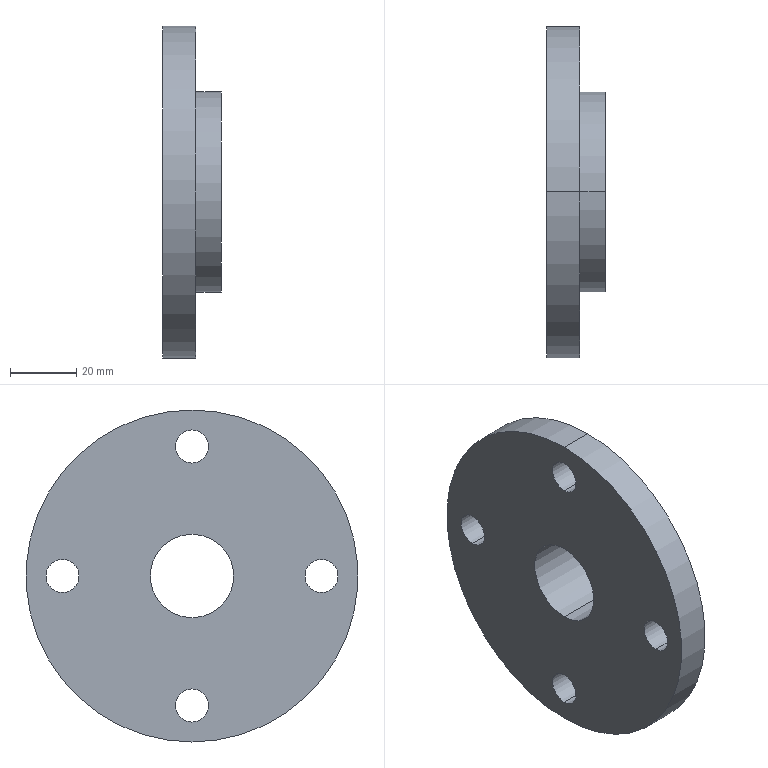Component | SolidWorks | FrontEndCap-1 | 1 solid | 17 faces | box 17.71 x 100 x 100 mm | volume 88740 mm3 | cylinder 14 | plane 3 | commonest cylinder face diameters 10 x8 25.135 x2 60.457 x2 100 x2
build123d program:
from build123d import *

# Parameters (mm, degrees)
SKETCH3_R          = 5
CUT_EXTRUDE1_DEPTH = 10


with BuildPart() as part:
    # Sketch2 → Revolve1 (revolve)
    with BuildSketch(Plane.ZY.offset(15), mode=Mode.PRIVATE) as revolve1_sk:
        Polygon((12.303, 200), (2.303, 200), (2.303, 180.229), (-5.405, 180.229), (-5.405, 162.567), (12.303, 162.567), align=None)
    revolve(revolve1_sk.sketch.rotate(Axis((-15, 150, 63.319), (0, 0, -1)), 90), axis=Axis((-15, 150, 63.319), (0, 0, -1)))

    # Sketch3 → Cut-Extrude1 (cut)
    with BuildSketch(Plane.XY.offset(12.303)):
        with Locations((24, 150)):
            Circle(SKETCH3_R)
        with Locations((-15, 111)):
            Circle(SKETCH3_R)
        with Locations((-54, 150)):
            Circle(SKETCH3_R)
        with Locations((-15, 189)):
            Circle(SKETCH3_R)
    extrude(amount=-CUT_EXTRUDE1_DEPTH, mode=Mode.SUBTRACT)


solid = part.part

# Placed as in the assembly
solid = solid.moved(Location((-122.697, 0, 0), (0, -90, 0)))
STEP:
#1=COLOUR_RGB('',0.7922,0.8196,0.9333);
#2=FILL_AREA_STYLE_COLOUR('',#1);
#3=FILL_AREA_STYLE('',(#2));
#4=SURFACE_STYLE_FILL_AREA(#3);
#5=SURFACE_SIDE_STYLE('',(#4));
#6=SURFACE_STYLE_USAGE(.BOTH.,#5);
#7=PRESENTATION_STYLE_ASSIGNMENT((#6));
#8=CARTESIAN_POINT('',(-4.921,5.906,0.748));
#9=VERTEX_POINT('',#8);
#10=CARTESIAN_POINT('',(-4.921,5.906,1.142));
#11=VERTEX_POINT('',#10);
#12=CARTESIAN_POINT('',(-4.921,5.906,0.9449));
#13=DIRECTION('',(-1.,0.,0.));
#14=DIRECTION('',(0.,0.,1.));
#15=AXIS2_PLACEMENT_3D('',#12,#13,#14);
#16=CIRCLE('',#15,0.1969);
#17=EDGE_CURVE('',#9,#11,#16,.T.);
#18=ORIENTED_EDGE('',*,*,#17,.F.);
#19=CARTESIAN_POINT('',(-5.315,5.906,0.748));
#20=VERTEX_POINT('',#19);
#21=CARTESIAN_POINT('',(-4.921,5.906,0.748));
#22=DIRECTION('',(-1.,0.,0.));
#23=VECTOR('',#22,39.37);
#24=LINE('',#21,#23);
#25=EDGE_CURVE('',#9,#20,#24,.T.);
#26=ORIENTED_EDGE('',*,*,#25,.T.);
#27=CARTESIAN_POINT('',(-5.315,5.906,1.142));
#28=VERTEX_POINT('',#27);
#29=CARTESIAN_POINT('',(-5.315,5.906,0.9449));
#30=DIRECTION('',(-1.,0.,0.));
#31=DIRECTION('',(0.,0.,1.));
#32=AXIS2_PLACEMENT_3D('',#29,#30,#31);
#33=CIRCLE('',#32,0.1969);
#34=EDGE_CURVE('',#20,#28,#33,.T.);
#35=ORIENTED_EDGE('',*,*,#34,.T.);
#36=CARTESIAN_POINT('',(-4.921,5.906,1.142));
#37=DIRECTION('',(-1.,0.,0.));
#38=VECTOR('',#37,39.37);
#39=LINE('',#36,#38);
#40=EDGE_CURVE('',#11,#28,#39,.T.);
#41=ORIENTED_EDGE('',*,*,#40,.F.);
#42=EDGE_LOOP('',(#18,#26,#35,#41));
#43=FACE_OUTER_BOUND('',#42,.T.);
#44=CARTESIAN_POINT('',(-4.921,5.906,0.9449));
#45=DIRECTION('',(-1.,0.,0.));
#46=DIRECTION('',(0.,0.,1.));
#47=AXIS2_PLACEMENT_3D('',#44,#45,#46);
#48=CYLINDRICAL_SURFACE('',#47,0.1969);
#49=ADVANCED_FACE('',(#43),#48,.F.);
#50=CARTESIAN_POINT('',(-4.921,4.37,-0.7874));
#51=VERTEX_POINT('',#50);
#52=CARTESIAN_POINT('',(-4.921,4.37,-0.3937));
#53=VERTEX_POINT('',#52);
#54=CARTESIAN_POINT('',(-4.921,4.37,-0.5906));
#55=DIRECTION('',(-1.,0.,0.));
#56=DIRECTION('',(0.,0.,1.));
#57=AXIS2_PLACEMENT_3D('',#54,#55,#56);
#58=CIRCLE('',#57,0.1969);
#59=EDGE_CURVE('',#51,#53,#58,.T.);
#60=ORIENTED_EDGE('',*,*,#59,.F.);
#61=CARTESIAN_POINT('',(-5.315,4.37,-0.7874));
#62=VERTEX_POINT('',#61);
#63=CARTESIAN_POINT('',(-4.921,4.37,-0.7874));
#64=DIRECTION('',(-1.,0.,0.));
#65=VECTOR('',#64,39.37);
#66=LINE('',#63,#65);
#67=EDGE_CURVE('',#51,#62,#66,.T.);
#68=ORIENTED_EDGE('',*,*,#67,.T.);
#69=CARTESIAN_POINT('',(-5.315,4.37,-0.3937));
#70=VERTEX_POINT('',#69);
#71=CARTESIAN_POINT('',(-5.315,4.37,-0.5906));
#72=DIRECTION('',(-1.,0.,0.));
#73=DIRECTION('',(0.,0.,1.));
#74=AXIS2_PLACEMENT_3D('',#71,#72,#73);
#75=CIRCLE('',#74,0.1969);
#76=EDGE_CURVE('',#62,#70,#75,.T.);
#77=ORIENTED_EDGE('',*,*,#76,.T.);
#78=CARTESIAN_POINT('',(-4.921,4.37,-0.3937));
#79=DIRECTION('',(-1.,0.,0.));
#80=VECTOR('',#79,39.37);
#81=LINE('',#78,#80);
#82=EDGE_CURVE('',#53,#70,#81,.T.);
#83=ORIENTED_EDGE('',*,*,#82,.F.);
#84=EDGE_LOOP('',(#60,#68,#77,#83));
#85=FACE_OUTER_BOUND('',#84,.T.);
#86=CARTESIAN_POINT('',(-4.921,4.37,-0.5906));
#87=DIRECTION('',(-1.,0.,0.));
#88=DIRECTION('',(0.,0.,1.));
#89=AXIS2_PLACEMENT_3D('',#86,#87,#88);
#90=CYLINDRICAL_SURFACE('',#89,0.1969);
#91=ADVANCED_FACE('',(#85),#90,.F.);
#92=CARTESIAN_POINT('',(-4.921,5.906,-2.323));
#93=VERTEX_POINT('',#92);
#94=CARTESIAN_POINT('',(-4.921,5.906,-1.929));
#95=VERTEX_POINT('',#94);
#96=CARTESIAN_POINT('',(-4.921,5.906,-2.126));
#97=DIRECTION('',(-1.,0.,0.));
#98=DIRECTION('',(0.,0.,1.));
#99=AXIS2_PLACEMENT_3D('',#96,#97,#98);
#100=CIRCLE('',#99,0.1969);
#101=EDGE_CURVE('',#93,#95,#100,.T.);
#102=ORIENTED_EDGE('',*,*,#101,.F.);
#103=CARTESIAN_POINT('',(-5.315,5.906,-2.323));
#104=VERTEX_POINT('',#103);
#105=CARTESIAN_POINT('',(-4.921,5.906,-2.323));
#106=DIRECTION('',(-1.,0.,0.));
#107=VECTOR('',#106,39.37);
#108=LINE('',#105,#107);
#109=EDGE_CURVE('',#93,#104,#108,.T.);
#110=ORIENTED_EDGE('',*,*,#109,.T.);
#111=CARTESIAN_POINT('',(-5.315,5.906,-1.929));
#112=VERTEX_POINT('',#111);
#113=CARTESIAN_POINT('',(-5.315,5.906,-2.126));
#114=DIRECTION('',(-1.,0.,0.));
#115=DIRECTION('',(0.,0.,1.));
#116=AXIS2_PLACEMENT_3D('',#113,#114,#115);
#117=CIRCLE('',#116,0.1969);
#118=EDGE_CURVE('',#104,#112,#117,.T.);
#119=ORIENTED_EDGE('',*,*,#118,.T.);
#120=CARTESIAN_POINT('',(-4.921,5.906,-1.929));
#121=DIRECTION('',(-1.,0.,0.));
#122=VECTOR('',#121,39.37);
#123=LINE('',#120,#122);
#124=EDGE_CURVE('',#95,#112,#123,.T.);
#125=ORIENTED_EDGE('',*,*,#124,.F.);
#126=EDGE_LOOP('',(#102,#110,#119,#125));
#127=FACE_OUTER_BOUND('',#126,.T.);
#128=CARTESIAN_POINT('',(-4.921,5.906,-2.126));
#129=DIRECTION('',(-1.,0.,0.));
#130=DIRECTION('',(0.,0.,1.));
#131=AXIS2_PLACEMENT_3D('',#128,#129,#130);
#132=CYLINDRICAL_SURFACE('',#131,0.1969);
#133=ADVANCED_FACE('',(#127),#132,.F.);
#134=CARTESIAN_POINT('',(-4.921,7.441,-0.7874));
#135=VERTEX_POINT('',#134);
#136=CARTESIAN_POINT('',(-4.921,7.441,-0.3937));
#137=VERTEX_POINT('',#136);
#138=CARTESIAN_POINT('',(-4.921,7.441,-0.5906));
#139=DIRECTION('',(-1.,0.,0.));
#140=DIRECTION('',(0.,0.,1.));
#141=AXIS2_PLACEMENT_3D('',#138,#139,#140);
#142=CIRCLE('',#141,0.1969);
#143=EDGE_CURVE('',#135,#137,#142,.T.);
#144=ORIENTED_EDGE('',*,*,#143,.F.);
#145=CARTESIAN_POINT('',(-5.315,7.441,-0.7874));
#146=VERTEX_POINT('',#145);
#147=CARTESIAN_POINT('',(-4.921,7.441,-0.7874));
#148=DIRECTION('',(-1.,0.,0.));
#149=VECTOR('',#148,39.37);
#150=LINE('',#147,#149);
#151=EDGE_CURVE('',#135,#146,#150,.T.);
#152=ORIENTED_EDGE('',*,*,#151,.T.);
#153=CARTESIAN_POINT('',(-5.315,7.441,-0.3937));
#154=VERTEX_POINT('',#153);
#155=CARTESIAN_POINT('',(-5.315,7.441,-0.5906));
#156=DIRECTION('',(-1.,0.,0.));
#157=DIRECTION('',(0.,0.,1.));
#158=AXIS2_PLACEMENT_3D('',#155,#156,#157);
#159=CIRCLE('',#158,0.1969);
#160=EDGE_CURVE('',#146,#154,#159,.T.);
#161=ORIENTED_EDGE('',*,*,#160,.T.);
#162=CARTESIAN_POINT('',(-4.921,7.441,-0.3937));
#163=DIRECTION('',(-1.,0.,0.));
#164=VECTOR('',#163,39.37);
#165=LINE('',#162,#164);
#166=EDGE_CURVE('',#137,#154,#165,.T.);
#167=ORIENTED_EDGE('',*,*,#166,.F.);
#168=EDGE_LOOP('',(#144,#152,#161,#167));
#169=FACE_OUTER_BOUND('',#168,.T.);
#170=CARTESIAN_POINT('',(-4.921,7.441,-0.5906));
#171=DIRECTION('',(-1.,0.,0.));
#172=DIRECTION('',(0.,0.,1.));
#173=AXIS2_PLACEMENT_3D('',#170,#171,#172);
#174=CYLINDRICAL_SURFACE('',#173,0.1969);
#175=ADVANCED_FACE('',(#169),#174,.F.);
#176=CARTESIAN_POINT('',(-4.618,5.906,-1.085));
#177=VERTEX_POINT('',#176);
#178=CARTESIAN_POINT('',(-4.618,5.906,-0.09578));
#179=VERTEX_POINT('',#178);
#180=CARTESIAN_POINT('',(-4.618,5.906,-0.5906));
#181=DIRECTION('',(-1.,0.,0.));
#182=DIRECTION('',(0.,0.,1.));
#183=AXIS2_PLACEMENT_3D('',#180,#181,#182);
#184=CIRCLE('',#183,0.4948);
#185=EDGE_CURVE('',#177,#179,#184,.T.);
#186=ORIENTED_EDGE('',*,*,#185,.F.);
#187=CARTESIAN_POINT('',(-5.315,5.906,-1.085));
#188=VERTEX_POINT('',#187);
#189=CARTESIAN_POINT('',(-7.323,5.906,-1.085));
#190=DIRECTION('',(-1.,0.,0.));
#191=VECTOR('',#190,39.37);
#192=LINE('',#189,#191);
#193=EDGE_CURVE('',#177,#188,#192,.T.);
#194=ORIENTED_EDGE('',*,*,#193,.T.);
#195=CARTESIAN_POINT('',(-5.315,5.906,-0.09578));
#196=VERTEX_POINT('',#195);
#197=CARTESIAN_POINT('',(-5.315,5.906,-0.5906));
#198=DIRECTION('',(-1.,0.,0.));
#199=DIRECTION('',(0.,0.,1.));
#200=AXIS2_PLACEMENT_3D('',#197,#198,#199);
#201=CIRCLE('',#200,0.4948);
#202=EDGE_CURVE('',#188,#196,#201,.T.);
#203=ORIENTED_EDGE('',*,*,#202,.T.);
#204=CARTESIAN_POINT('',(-7.323,5.906,-0.09578));
#205=DIRECTION('',(-1.,0.,0.));
#206=VECTOR('',#205,39.37);
#207=LINE('',#204,#206);
#208=EDGE_CURVE('',#179,#196,#207,.T.);
#209=ORIENTED_EDGE('',*,*,#208,.F.);
#210=EDGE_LOOP('',(#186,#194,#203,#209));
#211=FACE_OUTER_BOUND('',#210,.T.);
#212=CARTESIAN_POINT('',(-7.323,5.906,-0.5906));
#213=DIRECTION('',(-1.,0.,0.));
#214=DIRECTION('',(0.,0.,1.));
#215=AXIS2_PLACEMENT_3D('',#212,#213,#214);
#216=CYLINDRICAL_SURFACE('',#215,0.4948);
#217=ADVANCED_FACE('',(#211),#216,.F.);
#218=CARTESIAN_POINT('',(-4.618,5.906,0.5996));
#219=VERTEX_POINT('',#218);
#220=CARTESIAN_POINT('',(-4.618,5.906,-1.781));
#221=VERTEX_POINT('',#220);
#222=CARTESIAN_POINT('',(-4.618,5.906,-0.5906));
#223=DIRECTION('',(-1.,0.,0.));
#224=DIRECTION('',(0.,0.,1.));
#225=AXIS2_PLACEMENT_3D('',#222,#223,#224);
#226=CIRCLE('',#225,1.19);
#227=EDGE_CURVE('',#219,#221,#226,.T.);
#228=ORIENTED_EDGE('',*,*,#227,.T.);
#229=CARTESIAN_POINT('',(-4.921,5.906,-1.781));
#230=VERTEX_POINT('',#229);
#231=CARTESIAN_POINT('',(-7.323,5.906,-1.781));
#232=DIRECTION('',(-1.,0.,0.));
#233=VECTOR('',#232,39.37);
#234=LINE('',#231,#233);
#235=EDGE_CURVE('',#221,#230,#234,.T.);
#236=ORIENTED_EDGE('',*,*,#235,.T.);
#237=CARTESIAN_POINT('',(-4.921,5.906,0.5996));
#238=VERTEX_POINT('',#237);
#239=CARTESIAN_POINT('',(-4.921,5.906,-0.5906));
#240=DIRECTION('',(-1.,0.,0.));
#241=DIRECTION('',(0.,0.,1.));
#242=AXIS2_PLACEMENT_3D('',#239,#240,#241);
#243=CIRCLE('',#242,1.19);
#244=EDGE_CURVE('',#238,#230,#243,.T.);
#245=ORIENTED_EDGE('',*,*,#244,.F.);
#246=CARTESIAN_POINT('',(-7.323,5.906,0.5996));
#247=DIRECTION('',(-1.,0.,0.));
#248=VECTOR('',#247,39.37);
#249=LINE('',#246,#248);
#250=EDGE_CURVE('',#219,#238,#249,.T.);
#251=ORIENTED_EDGE('',*,*,#250,.F.);
#252=EDGE_LOOP('',(#228,#236,#245,#251));
#253=FACE_OUTER_BOUND('',#252,.T.);
#254=CARTESIAN_POINT('',(-7.323,5.906,-0.5906));
#255=DIRECTION('',(-1.,0.,0.));
#256=DIRECTION('',(0.,0.,1.));
#257=AXIS2_PLACEMENT_3D('',#254,#255,#256);
#258=CYLINDRICAL_SURFACE('',#257,1.19);
#259=ADVANCED_FACE('',(#253),#258,.T.);
#260=CARTESIAN_POINT('',(-4.921,5.906,1.378));
#261=VERTEX_POINT('',#260);
#262=CARTESIAN_POINT('',(-4.921,5.906,-2.559));
#263=VERTEX_POINT('',#262);
#264=CARTESIAN_POINT('',(-4.921,5.906,-0.5906));
#265=DIRECTION('',(-1.,0.,0.));
#266=DIRECTION('',(0.,0.,1.));
#267=AXIS2_PLACEMENT_3D('',#264,#265,#266);
#268=CIRCLE('',#267,1.969);
#269=EDGE_CURVE('',#261,#263,#268,.T.);
#270=ORIENTED_EDGE('',*,*,#269,.T.);
#271=CARTESIAN_POINT('',(-5.315,5.906,-2.559));
#272=VERTEX_POINT('',#271);
#273=CARTESIAN_POINT('',(-7.323,5.906,-2.559));
#274=DIRECTION('',(-1.,0.,0.));
#275=VECTOR('',#274,39.37);
#276=LINE('',#273,#275);
#277=EDGE_CURVE('',#263,#272,#276,.T.);
#278=ORIENTED_EDGE('',*,*,#277,.T.);
#279=CARTESIAN_POINT('',(-5.315,5.906,1.378));
#280=VERTEX_POINT('',#279);
#281=CARTESIAN_POINT('',(-5.315,5.906,-0.5906));
#282=DIRECTION('',(-1.,0.,0.));
#283=DIRECTION('',(0.,0.,1.));
#284=AXIS2_PLACEMENT_3D('',#281,#282,#283);
#285=CIRCLE('',#284,1.969);
#286=EDGE_CURVE('',#280,#272,#285,.T.);
#287=ORIENTED_EDGE('',*,*,#286,.F.);
#288=CARTESIAN_POINT('',(-7.323,5.906,1.378));
#289=DIRECTION('',(-1.,0.,0.));
#290=VECTOR('',#289,39.37);
#291=LINE('',#288,#290);
#292=EDGE_CURVE('',#261,#280,#291,.T.);
#293=ORIENTED_EDGE('',*,*,#292,.F.);
#294=EDGE_LOOP('',(#270,#278,#287,#293));
#295=FACE_OUTER_BOUND('',#294,.T.);
#296=CARTESIAN_POINT('',(-7.323,5.906,-0.5906));
#297=DIRECTION('',(-1.,0.,0.));
#298=DIRECTION('',(0.,0.,1.));
#299=AXIS2_PLACEMENT_3D('',#296,#297,#298);
#300=CYLINDRICAL_SURFACE('',#299,1.969);
#301=ADVANCED_FACE('',(#295),#300,.T.);
#302=CARTESIAN_POINT('',(-5.315,5.906,0.9449));
#303=DIRECTION('',(-1.,0.,0.));
#304=DIRECTION('',(0.,0.,1.));
#305=AXIS2_PLACEMENT_3D('',#302,#303,#304);
#306=CIRCLE('',#305,0.1969);
#307=EDGE_CURVE('',#28,#20,#306,.T.);
#308=ORIENTED_EDGE('',*,*,#307,.F.);
#309=ORIENTED_EDGE('',*,*,#34,.F.);
#310=EDGE_LOOP('',(#308,#309));
#311=FACE_BOUND('',#310,.T.);
#312=CARTESIAN_POINT('',(-5.315,4.37,-0.5906));
#313=DIRECTION('',(-1.,0.,0.));
#314=DIRECTION('',(0.,0.,1.));
#315=AXIS2_PLACEMENT_3D('',#312,#313,#314);
#316=CIRCLE('',#315,0.1969);
#317=EDGE_CURVE('',#70,#62,#316,.T.);
#318=ORIENTED_EDGE('',*,*,#317,.F.);
#319=ORIENTED_EDGE('',*,*,#76,.F.);
#320=EDGE_LOOP('',(#318,#319));
#321=FACE_BOUND('',#320,.T.);
#322=CARTESIAN_POINT('',(-5.315,5.906,-2.126));
#323=DIRECTION('',(-1.,0.,0.));
#324=DIRECTION('',(0.,0.,1.));
#325=AXIS2_PLACEMENT_3D('',#322,#323,#324);
#326=CIRCLE('',#325,0.1969);
#327=EDGE_CURVE('',#112,#104,#326,.T.);
#328=ORIENTED_EDGE('',*,*,#327,.F.);
#329=ORIENTED_EDGE('',*,*,#118,.F.);
#330=EDGE_LOOP('',(#328,#329));
#331=FACE_BOUND('',#330,.T.);
#332=CARTESIAN_POINT('',(-5.315,7.441,-0.5906));
#333=DIRECTION('',(-1.,0.,0.));
#334=DIRECTION('',(0.,0.,1.));
#335=AXIS2_PLACEMENT_3D('',#332,#333,#334);
#336=CIRCLE('',#335,0.1969);
#337=EDGE_CURVE('',#154,#146,#336,.T.);
#338=ORIENTED_EDGE('',*,*,#337,.F.);
#339=ORIENTED_EDGE('',*,*,#160,.F.);
#340=EDGE_LOOP('',(#338,#339));
#341=FACE_BOUND('',#340,.T.);
#342=ORIENTED_EDGE('',*,*,#286,.T.);
#343=CARTESIAN_POINT('',(-5.315,5.906,-0.5906));
#344=DIRECTION('',(-1.,0.,0.));
#345=DIRECTION('',(0.,0.,1.));
#346=AXIS2_PLACEMENT_3D('',#343,#344,#345);
#347=CIRCLE('',#346,1.969);
#348=EDGE_CURVE('',#272,#280,#347,.T.);
#349=ORIENTED_EDGE('',*,*,#348,.T.);
#350=EDGE_LOOP('',(#342,#349));
#351=FACE_OUTER_BOUND('',#350,.T.);
#352=CARTESIAN_POINT('',(-5.315,5.906,-0.5906));
#353=DIRECTION('',(-1.,0.,0.));
#354=DIRECTION('',(0.,0.,1.));
#355=AXIS2_PLACEMENT_3D('',#352,#353,#354);
#356=CIRCLE('',#355,0.4948);
#357=EDGE_CURVE('',#196,#188,#356,.T.);
#358=ORIENTED_EDGE('',*,*,#357,.F.);
#359=ORIENTED_EDGE('',*,*,#202,.F.);
#360=EDGE_LOOP('',(#358,#359));
#361=FACE_BOUND('',#360,.T.);
#362=CARTESIAN_POINT('',(-5.315,6.4,-0.5906));
#363=DIRECTION('',(-1.,0.,0.));
#364=DIRECTION('',(0.,0.,1.));
#365=AXIS2_PLACEMENT_3D('',#362,#363,#364);
#366=PLANE('',#365);
#367=ADVANCED_FACE('',(#311,#321,#331,#341,#351,#361),#366,.T.);
#368=ORIENTED_EDGE('',*,*,#277,.F.);
#369=CARTESIAN_POINT('',(-4.921,5.906,-0.5906));
#370=DIRECTION('',(-1.,0.,0.));
#371=DIRECTION('',(0.,0.,1.));
#372=AXIS2_PLACEMENT_3D('',#369,#370,#371);
#373=CIRCLE('',#372,1.969);
#374=EDGE_CURVE('',#263,#261,#373,.T.);
#375=ORIENTED_EDGE('',*,*,#374,.T.);
#376=ORIENTED_EDGE('',*,*,#292,.T.);
#377=ORIENTED_EDGE('',*,*,#348,.F.);
#378=EDGE_LOOP('',(#368,#375,#376,#377));
#379=FACE_OUTER_BOUND('',#378,.T.);
#380=CARTESIAN_POINT('',(-7.323,5.906,-0.5906));
#381=DIRECTION('',(-1.,0.,0.));
#382=DIRECTION('',(0.,0.,1.));
#383=AXIS2_PLACEMENT_3D('',#380,#381,#382);
#384=CYLINDRICAL_SURFACE('',#383,1.969);
#385=ADVANCED_FACE('',(#379),#384,.T.);
#386=CARTESIAN_POINT('',(-4.921,5.906,0.9449));
#387=DIRECTION('',(-1.,0.,0.));
#388=DIRECTION('',(0.,0.,1.));
#389=AXIS2_PLACEMENT_3D('',#386,#387,#388);
#390=CIRCLE('',#389,0.1969);
#391=EDGE_CURVE('',#11,#9,#390,.T.);
#392=ORIENTED_EDGE('',*,*,#391,.T.);
#393=ORIENTED_EDGE('',*,*,#17,.T.);
#394=EDGE_LOOP('',(#392,#393));
#395=FACE_BOUND('',#394,.T.);
#396=CARTESIAN_POINT('',(-4.921,4.37,-0.5906));
#397=DIRECTION('',(-1.,0.,0.));
#398=DIRECTION('',(0.,0.,1.));
#399=AXIS2_PLACEMENT_3D('',#396,#397,#398);
#400=CIRCLE('',#399,0.1969);
#401=EDGE_CURVE('',#53,#51,#400,.T.);
#402=ORIENTED_EDGE('',*,*,#401,.T.);
#403=ORIENTED_EDGE('',*,*,#59,.T.);
#404=EDGE_LOOP('',(#402,#403));
#405=FACE_BOUND('',#404,.T.);
#406=CARTESIAN_POINT('',(-4.921,5.906,-2.126));
#407=DIRECTION('',(-1.,0.,0.));
#408=DIRECTION('',(0.,0.,1.));
#409=AXIS2_PLACEMENT_3D('',#406,#407,#408);
#410=CIRCLE('',#409,0.1969);
#411=EDGE_CURVE('',#95,#93,#410,.T.);
#412=ORIENTED_EDGE('',*,*,#411,.T.);
#413=ORIENTED_EDGE('',*,*,#101,.T.);
#414=EDGE_LOOP('',(#412,#413));
#415=FACE_BOUND('',#414,.T.);
#416=CARTESIAN_POINT('',(-4.921,7.441,-0.5906));
#417=DIRECTION('',(-1.,0.,0.));
#418=DIRECTION('',(0.,0.,1.));
#419=AXIS2_PLACEMENT_3D('',#416,#417,#418);
#420=CIRCLE('',#419,0.1969);
#421=EDGE_CURVE('',#137,#135,#420,.T.);
#422=ORIENTED_EDGE('',*,*,#421,.T.);
#423=ORIENTED_EDGE('',*,*,#143,.T.);
#424=EDGE_LOOP('',(#422,#423));
#425=FACE_BOUND('',#424,.T.);
#426=ORIENTED_EDGE('',*,*,#244,.T.);
#427=CARTESIAN_POINT('',(-4.921,5.906,-0.5906));
#428=DIRECTION('',(-1.,0.,0.));
#429=DIRECTION('',(0.,0.,1.));
#430=AXIS2_PLACEMENT_3D('',#427,#428,#429);
#431=CIRCLE('',#430,1.19);
#432=EDGE_CURVE('',#230,#238,#431,.T.);
#433=ORIENTED_EDGE('',*,*,#432,.T.);
#434=EDGE_LOOP('',(#426,#433));
#435=FACE_BOUND('',#434,.T.);
#436=ORIENTED_EDGE('',*,*,#269,.F.);
#437=ORIENTED_EDGE('',*,*,#374,.F.);
#438=EDGE_LOOP('',(#436,#437));
#439=FACE_OUTER_BOUND('',#438,.T.);
#440=CARTESIAN_POINT('',(-4.921,7.874,-0.5906));
#441=DIRECTION('',(1.,0.,0.));
#442=DIRECTION('',(0.,-0.,-1.));
#443=AXIS2_PLACEMENT_3D('',#440,#441,#442);
#444=PLANE('',#443);
#445=ADVANCED_FACE('',(#395,#405,#415,#425,#435,#439),#444,.T.);
#446=ORIENTED_EDGE('',*,*,#235,.F.);
#447=CARTESIAN_POINT('',(-4.618,5.906,-0.5906));
#448=DIRECTION('',(-1.,0.,0.));
#449=DIRECTION('',(0.,0.,1.));
#450=AXIS2_PLACEMENT_3D('',#447,#448,#449);
#451=CIRCLE('',#450,1.19);
#452=EDGE_CURVE('',#221,#219,#451,.T.);
#453=ORIENTED_EDGE('',*,*,#452,.T.);
#454=ORIENTED_EDGE('',*,*,#250,.T.);
#455=ORIENTED_EDGE('',*,*,#432,.F.);
#456=EDGE_LOOP('',(#446,#453,#454,#455));
#457=FACE_OUTER_BOUND('',#456,.T.);
#458=CARTESIAN_POINT('',(-7.323,5.906,-0.5906));
#459=DIRECTION('',(-1.,0.,0.));
#460=DIRECTION('',(0.,0.,1.));
#461=AXIS2_PLACEMENT_3D('',#458,#459,#460);
#462=CYLINDRICAL_SURFACE('',#461,1.19);
#463=ADVANCED_FACE('',(#457),#462,.T.);
#464=CARTESIAN_POINT('',(-4.618,5.906,-0.5906));
#465=DIRECTION('',(-1.,0.,0.));
#466=DIRECTION('',(0.,0.,1.));
#467=AXIS2_PLACEMENT_3D('',#464,#465,#466);
#468=CIRCLE('',#467,0.4948);
#469=EDGE_CURVE('',#179,#177,#468,.T.);
#470=ORIENTED_EDGE('',*,*,#469,.T.);
#471=ORIENTED_EDGE('',*,*,#185,.T.);
#472=EDGE_LOOP('',(#470,#471));
#473=FACE_BOUND('',#472,.T.);
#474=ORIENTED_EDGE('',*,*,#227,.F.);
#475=ORIENTED_EDGE('',*,*,#452,.F.);
#476=EDGE_LOOP('',(#474,#475));
#477=FACE_OUTER_BOUND('',#476,.T.);
#478=CARTESIAN_POINT('',(-4.618,7.096,-0.5906));
#479=DIRECTION('',(1.,0.,0.));
#480=DIRECTION('',(0.,-0.,-1.));
#481=AXIS2_PLACEMENT_3D('',#478,#479,#480);
#482=PLANE('',#481);
#483=ADVANCED_FACE('',(#473,#477),#482,.T.);
#484=ORIENTED_EDGE('',*,*,#193,.F.);
#485=ORIENTED_EDGE('',*,*,#469,.F.);
#486=ORIENTED_EDGE('',*,*,#208,.T.);
#487=ORIENTED_EDGE('',*,*,#357,.T.);
#488=EDGE_LOOP('',(#484,#485,#486,#487));
#489=FACE_OUTER_BOUND('',#488,.T.);
#490=CARTESIAN_POINT('',(-7.323,5.906,-0.5906));
#491=DIRECTION('',(-1.,0.,0.));
#492=DIRECTION('',(0.,0.,1.));
#493=AXIS2_PLACEMENT_3D('',#490,#491,#492);
#494=CYLINDRICAL_SURFACE('',#493,0.4948);
#495=ADVANCED_FACE('',(#489),#494,.F.);
#496=ORIENTED_EDGE('',*,*,#151,.F.);
#497=ORIENTED_EDGE('',*,*,#421,.F.);
#498=ORIENTED_EDGE('',*,*,#166,.T.);
#499=ORIENTED_EDGE('',*,*,#337,.T.);
#500=EDGE_LOOP('',(#496,#497,#498,#499));
#501=FACE_OUTER_BOUND('',#500,.T.);
#502=CARTESIAN_POINT('',(-4.921,7.441,-0.5906));
#503=DIRECTION('',(-1.,0.,0.));
#504=DIRECTION('',(0.,0.,1.));
#505=AXIS2_PLACEMENT_3D('',#502,#503,#504);
#506=CYLINDRICAL_SURFACE('',#505,0.1969);
#507=ADVANCED_FACE('',(#501),#506,.F.);
#508=ORIENTED_EDGE('',*,*,#109,.F.);
#509=ORIENTED_EDGE('',*,*,#411,.F.);
#510=ORIENTED_EDGE('',*,*,#124,.T.);
#511=ORIENTED_EDGE('',*,*,#327,.T.);
#512=EDGE_LOOP('',(#508,#509,#510,#511));
#513=FACE_OUTER_BOUND('',#512,.T.);
#514=CARTESIAN_POINT('',(-4.921,5.906,-2.126));
#515=DIRECTION('',(-1.,0.,0.));
#516=DIRECTION('',(0.,0.,1.));
#517=AXIS2_PLACEMENT_3D('',#514,#515,#516);
#518=CYLINDRICAL_SURFACE('',#517,0.1969);
#519=ADVANCED_FACE('',(#513),#518,.F.);
#520=ORIENTED_EDGE('',*,*,#67,.F.);
#521=ORIENTED_EDGE('',*,*,#401,.F.);
#522=ORIENTED_EDGE('',*,*,#82,.T.);
#523=ORIENTED_EDGE('',*,*,#317,.T.);
#524=EDGE_LOOP('',(#520,#521,#522,#523));
#525=FACE_OUTER_BOUND('',#524,.T.);
#526=CARTESIAN_POINT('',(-4.921,4.37,-0.5906));
#527=DIRECTION('',(-1.,0.,0.));
#528=DIRECTION('',(0.,0.,1.));
#529=AXIS2_PLACEMENT_3D('',#526,#527,#528);
#530=CYLINDRICAL_SURFACE('',#529,0.1969);
#531=ADVANCED_FACE('',(#525),#530,.F.);
#532=ORIENTED_EDGE('',*,*,#25,.F.);
#533=ORIENTED_EDGE('',*,*,#391,.F.);
#534=ORIENTED_EDGE('',*,*,#40,.T.);
#535=ORIENTED_EDGE('',*,*,#307,.T.);
#536=EDGE_LOOP('',(#532,#533,#534,#535));
#537=FACE_OUTER_BOUND('',#536,.T.);
#538=CARTESIAN_POINT('',(-4.921,5.906,0.9449));
#539=DIRECTION('',(-1.,0.,0.));
#540=DIRECTION('',(0.,0.,1.));
#541=AXIS2_PLACEMENT_3D('',#538,#539,#540);
#542=CYLINDRICAL_SURFACE('',#541,0.1969);
#543=ADVANCED_FACE('',(#537),#542,.F.);
#544=CLOSED_SHELL('',(#49,#91,#133,#175,#217,#259,#301,#367,#385,#445,#463,#483,#495,#507,#519,#531,#543));
#545=MANIFOLD_SOLID_BREP('',#544);
#546=STYLED_ITEM('',(#7),#545);
#547=(LENGTH_UNIT()NAMED_UNIT(*)SI_UNIT($,.METRE.));
#548=LENGTH_MEASURE_WITH_UNIT(LENGTH_MEASURE(0.0254),#547);
#549=DIMENSIONAL_EXPONENTS(1.,0.,0.,0.,0.,0.,0.);
#550=(CONVERSION_BASED_UNIT('',#548)LENGTH_UNIT()NAMED_UNIT(#549));
#551=UNCERTAINTY_MEASURE_WITH_UNIT(LENGTH_MEASURE(0.00001),#550,'','');
#552=(NAMED_UNIT(*)PLANE_ANGLE_UNIT()SI_UNIT($,.RADIAN.));
#553=(NAMED_UNIT(*)SI_UNIT($,.STERADIAN.)SOLID_ANGLE_UNIT());
#554=(GEOMETRIC_REPRESENTATION_CONTEXT(3)GLOBAL_UNCERTAINTY_ASSIGNED_CONTEXT((#551))GLOBAL_UNIT_ASSIGNED_CONTEXT((#550,#552,#553))REPRESENTATION_CONTEXT('',''));
#555=MECHANICAL_DESIGN_GEOMETRIC_PRESENTATION_REPRESENTATION('',(#546),#554);
#556=PRESENTATION_LAYER_ASSIGNMENT('','',(#546));
#557=CARTESIAN_POINT('',(0.,0.,0.));
#558=DIRECTION('',(0.,0.,1.));
#559=DIRECTION('',(1.,0.,0.));
#560=AXIS2_PLACEMENT_3D('',#557,#558,#559);
#561=(LENGTH_UNIT()NAMED_UNIT(*)SI_UNIT($,.METRE.));
#562=LENGTH_MEASURE_WITH_UNIT(LENGTH_MEASURE(0.0254),#561);
#563=DIMENSIONAL_EXPONENTS(1.,0.,0.,0.,0.,0.,0.);
#564=(CONVERSION_BASED_UNIT('',#562)LENGTH_UNIT()NAMED_UNIT(#563));
#565=UNCERTAINTY_MEASURE_WITH_UNIT(LENGTH_MEASURE(0.00001),#564,'','');
#566=(NAMED_UNIT(*)PLANE_ANGLE_UNIT()SI_UNIT($,.RADIAN.));
#567=(NAMED_UNIT(*)SI_UNIT($,.STERADIAN.)SOLID_ANGLE_UNIT());
#568=(GEOMETRIC_REPRESENTATION_CONTEXT(3)GLOBAL_UNCERTAINTY_ASSIGNED_CONTEXT((#565))GLOBAL_UNIT_ASSIGNED_CONTEXT((#564,#566,#567))REPRESENTATION_CONTEXT('',''));
#569=ADVANCED_BREP_SHAPE_REPRESENTATION('',(#545,#560),#568);